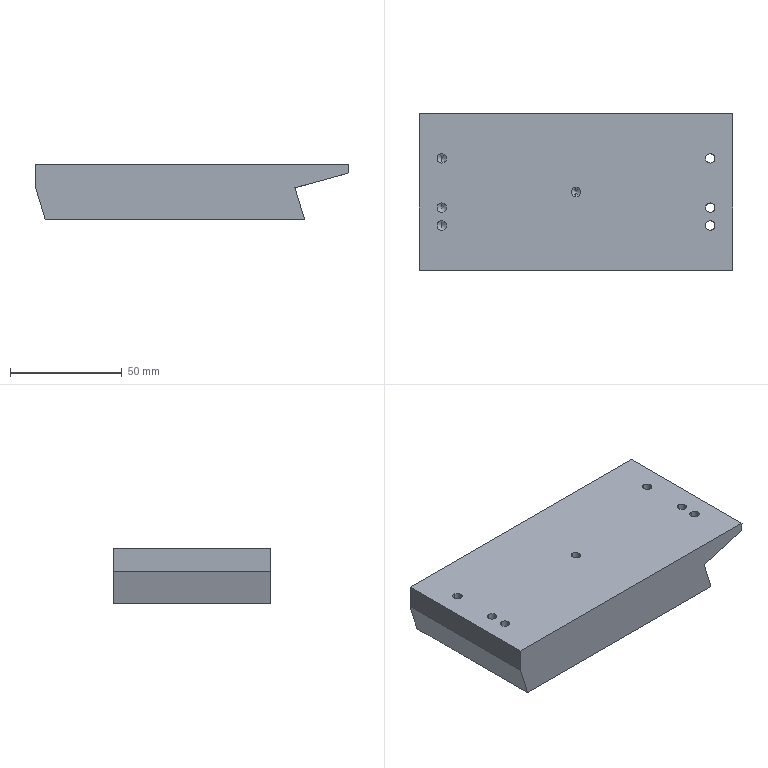Component | SolidWorks | FlatFeed-1_Part77-1 | 1 solid | 31 faces | box 140 x 70 x 25 mm | volume 214310 mm3 | cylinder 14 | plane 9 | cone 8 | commonest cylinder face diameters 4.2 x14
build123d program:
from build123d import *

# Parameters (mm, degrees)
EXTRUDE1_START        = -67.09
EXTRUDE1_DEPTH        = 70
M5_TAPPED_HOLE1_D     = 4.2
M5_TAPPED_HOLE1_DEPTH = 12.4
M5_TAPPED_HOLE1_TIP   = 1.262


with BuildPart() as part:
    # Sketch5 → Extrude1 (new body)
    with BuildSketch(Plane.XY.offset(EXTRUDE1_START)):
        Polygon((-988.993, 8051.776), (-988.993, 8047.776), (-964.993, 8041.132), (-969.382, 8026.776), (-853.382, 8026.776), (-848.993, 8041.132), (-848.993, 8051.776), align=None)
    extrude(amount=-EXTRUDE1_DEPTH)

    # M5 Tapped Hole1
    with Locations(Plane(origin=(0, 8051.776, 0), x_dir=(-1, 0, 0), z_dir=(0, 1, 0))):
        with Locations((978.993, -117.09), (978.993, -87.09), (858.993, -87.09), (858.993, -117.09), (978.993, -109.09), (918.993, -102.09), (858.993, -109.09)):
            Hole(M5_TAPPED_HOLE1_D / 2, depth=M5_TAPPED_HOLE1_DEPTH)
            with Locations((0, 0, -(M5_TAPPED_HOLE1_DEPTH + M5_TAPPED_HOLE1_TIP / 2))):  # 118° drill point
                Cone(0, M5_TAPPED_HOLE1_D / 2, M5_TAPPED_HOLE1_TIP, mode=Mode.SUBTRACT)


solid = part.part

# Placed as in the assembly
solid = solid.moved(Location((-740.399, -116.087, -7280.776), (-90, 0, 180)))
STEP:
#1=CARTESIAN_POINT('',(9.393,-9.097,30.088));
#2=VERTEX_POINT('',#1);
#3=CARTESIAN_POINT('',(9.393,-9.263,30.088));
#4=VERTEX_POINT('',#3);
#5=CARTESIAN_POINT('',(9.393,-9.097,30.088));
#6=CARTESIAN_POINT('',(9.559,-9.097,30.134));
#7=CARTESIAN_POINT('',(9.559,-9.263,30.134));
#8=CARTESIAN_POINT('',(9.393,-9.263,30.088));
#9=(BOUNDED_CURVE()B_SPLINE_CURVE(3,(#5,#6,#7,#8),.UNSPECIFIED.,.F.,.T.)B_SPLINE_CURVE_WITH_KNOTS((4,4),(4.712,7.854),.UNSPECIFIED.)CURVE()GEOMETRIC_REPRESENTATION_ITEM()RATIONAL_B_SPLINE_CURVE((1.,0.3333,0.3333,1.))REPRESENTATION_ITEM(''));
#10=EDGE_CURVE('',#2,#4,#9,.T.);
#11=ORIENTED_EDGE('',*,*,#10,.T.);
#12=CARTESIAN_POINT('',(9.393,-9.263,30.354));
#13=VERTEX_POINT('',#12);
#14=CARTESIAN_POINT('',(9.393,-9.263,30.354));
#15=DIRECTION('',(-0.,0.,1.));
#16=VECTOR('',#15,39.37);
#17=LINE('',#14,#16);
#18=EDGE_CURVE('',#4,#13,#17,.T.);
#19=ORIENTED_EDGE('',*,*,#18,.T.);
#20=CARTESIAN_POINT('',(9.393,-9.097,30.354));
#21=VERTEX_POINT('',#20);
#22=CARTESIAN_POINT('',(9.393,-9.18,30.354));
#23=DIRECTION('',(-0.,0.,1.));
#24=DIRECTION('',(0.,1.,0.));
#25=AXIS2_PLACEMENT_3D('',#22,#23,#24);
#26=CIRCLE('',#25,0.08268);
#27=EDGE_CURVE('',#13,#21,#26,.T.);
#28=ORIENTED_EDGE('',*,*,#27,.T.);
#29=CARTESIAN_POINT('',(9.393,-9.097,30.354));
#30=DIRECTION('',(-0.,0.,1.));
#31=VECTOR('',#30,39.37);
#32=LINE('',#29,#31);
#33=EDGE_CURVE('',#2,#21,#32,.T.);
#34=ORIENTED_EDGE('',*,*,#33,.F.);
#35=EDGE_LOOP('',(#11,#19,#28,#34));
#36=FACE_OUTER_BOUND('',#35,.T.);
#37=CARTESIAN_POINT('',(9.393,-9.18,30.354));
#38=DIRECTION('',(-0.,0.,1.));
#39=DIRECTION('',(0.,1.,0.));
#40=AXIS2_PLACEMENT_3D('',#37,#38,#39);
#41=CYLINDRICAL_SURFACE('',#40,0.08268);
#42=ADVANCED_FACE('',(#36),#41,.F.);
#43=CARTESIAN_POINT('',(9.393,-7.916,30.088));
#44=VERTEX_POINT('',#43);
#45=CARTESIAN_POINT('',(9.393,-8.082,30.088));
#46=VERTEX_POINT('',#45);
#47=CARTESIAN_POINT('',(9.393,-7.916,30.088));
#48=CARTESIAN_POINT('',(9.559,-7.916,30.134));
#49=CARTESIAN_POINT('',(9.559,-8.082,30.134));
#50=CARTESIAN_POINT('',(9.393,-8.082,30.088));
#51=(BOUNDED_CURVE()B_SPLINE_CURVE(3,(#47,#48,#49,#50),.UNSPECIFIED.,.F.,.T.)B_SPLINE_CURVE_WITH_KNOTS((4,4),(4.712,7.854),.UNSPECIFIED.)CURVE()GEOMETRIC_REPRESENTATION_ITEM()RATIONAL_B_SPLINE_CURVE((1.,0.3333,0.3333,1.))REPRESENTATION_ITEM(''));
#52=EDGE_CURVE('',#44,#46,#51,.T.);
#53=ORIENTED_EDGE('',*,*,#52,.T.);
#54=CARTESIAN_POINT('',(9.393,-8.082,30.354));
#55=VERTEX_POINT('',#54);
#56=CARTESIAN_POINT('',(9.393,-8.082,30.354));
#57=DIRECTION('',(-0.,0.,1.));
#58=VECTOR('',#57,39.37);
#59=LINE('',#56,#58);
#60=EDGE_CURVE('',#46,#55,#59,.T.);
#61=ORIENTED_EDGE('',*,*,#60,.T.);
#62=CARTESIAN_POINT('',(9.393,-7.916,30.354));
#63=VERTEX_POINT('',#62);
#64=CARTESIAN_POINT('',(9.393,-7.999,30.354));
#65=DIRECTION('',(-0.,0.,1.));
#66=DIRECTION('',(0.,1.,0.));
#67=AXIS2_PLACEMENT_3D('',#64,#65,#66);
#68=CIRCLE('',#67,0.08268);
#69=EDGE_CURVE('',#55,#63,#68,.T.);
#70=ORIENTED_EDGE('',*,*,#69,.T.);
#71=CARTESIAN_POINT('',(9.393,-7.916,30.354));
#72=DIRECTION('',(-0.,0.,1.));
#73=VECTOR('',#72,39.37);
#74=LINE('',#71,#73);
#75=EDGE_CURVE('',#44,#63,#74,.T.);
#76=ORIENTED_EDGE('',*,*,#75,.F.);
#77=EDGE_LOOP('',(#53,#61,#70,#76));
#78=FACE_OUTER_BOUND('',#77,.T.);
#79=CARTESIAN_POINT('',(9.393,-7.999,30.354));
#80=DIRECTION('',(-0.,0.,1.));
#81=DIRECTION('',(0.,1.,0.));
#82=AXIS2_PLACEMENT_3D('',#79,#80,#81);
#83=CYLINDRICAL_SURFACE('',#82,0.08268);
#84=ADVANCED_FACE('',(#78),#83,.F.);
#85=CARTESIAN_POINT('',(4.669,-8.082,29.866));
#86=VERTEX_POINT('',#85);
#87=CARTESIAN_POINT('',(4.669,-7.916,29.866));
#88=VERTEX_POINT('',#87);
#89=CARTESIAN_POINT('',(4.669,-7.999,29.866));
#90=DIRECTION('',(-0.,0.,1.));
#91=DIRECTION('',(0.,1.,0.));
#92=AXIS2_PLACEMENT_3D('',#89,#90,#91);
#93=CIRCLE('',#92,0.08268);
#94=EDGE_CURVE('',#86,#88,#93,.T.);
#95=ORIENTED_EDGE('',*,*,#94,.F.);
#96=CARTESIAN_POINT('',(4.669,-8.082,30.354));
#97=VERTEX_POINT('',#96);
#98=CARTESIAN_POINT('',(4.669,-8.082,30.354));
#99=DIRECTION('',(-0.,0.,1.));
#100=VECTOR('',#99,39.37);
#101=LINE('',#98,#100);
#102=EDGE_CURVE('',#86,#97,#101,.T.);
#103=ORIENTED_EDGE('',*,*,#102,.T.);
#104=CARTESIAN_POINT('',(4.669,-7.916,30.354));
#105=VERTEX_POINT('',#104);
#106=CARTESIAN_POINT('',(4.669,-7.999,30.354));
#107=DIRECTION('',(-0.,0.,1.));
#108=DIRECTION('',(0.,1.,0.));
#109=AXIS2_PLACEMENT_3D('',#106,#107,#108);
#110=CIRCLE('',#109,0.08268);
#111=EDGE_CURVE('',#97,#105,#110,.T.);
#112=ORIENTED_EDGE('',*,*,#111,.T.);
#113=CARTESIAN_POINT('',(4.669,-7.916,30.354));
#114=DIRECTION('',(-0.,0.,1.));
#115=VECTOR('',#114,39.37);
#116=LINE('',#113,#115);
#117=EDGE_CURVE('',#88,#105,#116,.T.);
#118=ORIENTED_EDGE('',*,*,#117,.F.);
#119=EDGE_LOOP('',(#95,#103,#112,#118));
#120=FACE_OUTER_BOUND('',#119,.T.);
#121=CARTESIAN_POINT('',(4.669,-7.999,30.354));
#122=DIRECTION('',(-0.,0.,1.));
#123=DIRECTION('',(0.,1.,0.));
#124=AXIS2_PLACEMENT_3D('',#121,#122,#123);
#125=CYLINDRICAL_SURFACE('',#124,0.08268);
#126=ADVANCED_FACE('',(#120),#125,.F.);
#127=CARTESIAN_POINT('',(4.669,-7.999,29.816));
#128=VERTEX_POINT('',#127);
#129=CARTESIAN_POINT('',(4.669,-7.916,29.866));
#130=DIRECTION('',(-0.,0.8572,0.515));
#131=VECTOR('',#130,39.37);
#132=LINE('',#129,#131);
#133=EDGE_CURVE('',#128,#88,#132,.T.);
#134=ORIENTED_EDGE('',*,*,#133,.F.);
#135=CARTESIAN_POINT('',(4.669,-8.082,29.866));
#136=DIRECTION('',(-0.,-0.8572,0.515));
#137=VECTOR('',#136,39.37);
#138=LINE('',#135,#137);
#139=EDGE_CURVE('',#128,#86,#138,.T.);
#140=ORIENTED_EDGE('',*,*,#139,.T.);
#141=ORIENTED_EDGE('',*,*,#94,.T.);
#142=EDGE_LOOP('',(#134,#140,#141));
#143=FACE_OUTER_BOUND('',#142,.T.);
#144=CARTESIAN_POINT('',(4.669,-7.999,29.866));
#145=DIRECTION('',(-0.,0.,1.));
#146=DIRECTION('',(0.,1.,0.));
#147=AXIS2_PLACEMENT_3D('',#144,#145,#146);
#148=CONICAL_SURFACE('',#147,0.08268,1.03);
#149=ADVANCED_FACE('',(#143),#148,.F.);
#150=CARTESIAN_POINT('',(4.669,-9.263,29.866));
#151=VERTEX_POINT('',#150);
#152=CARTESIAN_POINT('',(4.669,-9.097,29.866));
#153=VERTEX_POINT('',#152);
#154=CARTESIAN_POINT('',(4.669,-9.18,29.866));
#155=DIRECTION('',(-0.,0.,1.));
#156=DIRECTION('',(0.,1.,0.));
#157=AXIS2_PLACEMENT_3D('',#154,#155,#156);
#158=CIRCLE('',#157,0.08268);
#159=EDGE_CURVE('',#151,#153,#158,.T.);
#160=ORIENTED_EDGE('',*,*,#159,.F.);
#161=CARTESIAN_POINT('',(4.669,-9.263,30.354));
#162=VERTEX_POINT('',#161);
#163=CARTESIAN_POINT('',(4.669,-9.263,30.354));
#164=DIRECTION('',(-0.,0.,1.));
#165=VECTOR('',#164,39.37);
#166=LINE('',#163,#165);
#167=EDGE_CURVE('',#151,#162,#166,.T.);
#168=ORIENTED_EDGE('',*,*,#167,.T.);
#169=CARTESIAN_POINT('',(4.669,-9.097,30.354));
#170=VERTEX_POINT('',#169);
#171=CARTESIAN_POINT('',(4.669,-9.18,30.354));
#172=DIRECTION('',(-0.,0.,1.));
#173=DIRECTION('',(0.,1.,0.));
#174=AXIS2_PLACEMENT_3D('',#171,#172,#173);
#175=CIRCLE('',#174,0.08268);
#176=EDGE_CURVE('',#162,#170,#175,.T.);
#177=ORIENTED_EDGE('',*,*,#176,.T.);
#178=CARTESIAN_POINT('',(4.669,-9.097,30.354));
#179=DIRECTION('',(-0.,0.,1.));
#180=VECTOR('',#179,39.37);
#181=LINE('',#178,#180);
#182=EDGE_CURVE('',#153,#170,#181,.T.);
#183=ORIENTED_EDGE('',*,*,#182,.F.);
#184=EDGE_LOOP('',(#160,#168,#177,#183));
#185=FACE_OUTER_BOUND('',#184,.T.);
#186=CARTESIAN_POINT('',(4.669,-9.18,30.354));
#187=DIRECTION('',(-0.,0.,1.));
#188=DIRECTION('',(0.,1.,0.));
#189=AXIS2_PLACEMENT_3D('',#186,#187,#188);
#190=CYLINDRICAL_SURFACE('',#189,0.08268);
#191=ADVANCED_FACE('',(#185),#190,.F.);
#192=CARTESIAN_POINT('',(4.669,-9.18,29.816));
#193=VERTEX_POINT('',#192);
#194=CARTESIAN_POINT('',(4.669,-9.097,29.866));
#195=DIRECTION('',(-0.,0.8572,0.515));
#196=VECTOR('',#195,39.37);
#197=LINE('',#194,#196);
#198=EDGE_CURVE('',#193,#153,#197,.T.);
#199=ORIENTED_EDGE('',*,*,#198,.F.);
#200=CARTESIAN_POINT('',(4.669,-9.263,29.866));
#201=DIRECTION('',(-0.,-0.8572,0.515));
#202=VECTOR('',#201,39.37);
#203=LINE('',#200,#202);
#204=EDGE_CURVE('',#193,#151,#203,.T.);
#205=ORIENTED_EDGE('',*,*,#204,.T.);
#206=ORIENTED_EDGE('',*,*,#159,.T.);
#207=EDGE_LOOP('',(#199,#205,#206));
#208=FACE_OUTER_BOUND('',#207,.T.);
#209=CARTESIAN_POINT('',(4.669,-9.18,29.866));
#210=DIRECTION('',(-0.,0.,1.));
#211=DIRECTION('',(0.,1.,0.));
#212=AXIS2_PLACEMENT_3D('',#209,#210,#211);
#213=CONICAL_SURFACE('',#212,0.08268,1.03);
#214=ADVANCED_FACE('',(#208),#213,.F.);
#215=CARTESIAN_POINT('',(9.393,-8.783,30.088));
#216=VERTEX_POINT('',#215);
#217=CARTESIAN_POINT('',(9.393,-8.948,30.088));
#218=VERTEX_POINT('',#217);
#219=CARTESIAN_POINT('',(9.393,-8.783,30.088));
#220=CARTESIAN_POINT('',(9.559,-8.783,30.134));
#221=CARTESIAN_POINT('',(9.559,-8.948,30.134));
#222=CARTESIAN_POINT('',(9.393,-8.948,30.088));
#223=(BOUNDED_CURVE()B_SPLINE_CURVE(3,(#219,#220,#221,#222),.UNSPECIFIED.,.F.,.T.)B_SPLINE_CURVE_WITH_KNOTS((4,4),(4.712,7.854),.UNSPECIFIED.)CURVE()GEOMETRIC_REPRESENTATION_ITEM()RATIONAL_B_SPLINE_CURVE((1.,0.3333,0.3333,1.))REPRESENTATION_ITEM(''));
#224=EDGE_CURVE('',#216,#218,#223,.T.);
#225=ORIENTED_EDGE('',*,*,#224,.T.);
#226=CARTESIAN_POINT('',(9.393,-8.948,30.354));
#227=VERTEX_POINT('',#226);
#228=CARTESIAN_POINT('',(9.393,-8.948,30.354));
#229=DIRECTION('',(-0.,0.,1.));
#230=VECTOR('',#229,39.37);
#231=LINE('',#228,#230);
#232=EDGE_CURVE('',#218,#227,#231,.T.);
#233=ORIENTED_EDGE('',*,*,#232,.T.);
#234=CARTESIAN_POINT('',(9.393,-8.783,30.354));
#235=VERTEX_POINT('',#234);
#236=CARTESIAN_POINT('',(9.393,-8.865,30.354));
#237=DIRECTION('',(-0.,0.,1.));
#238=DIRECTION('',(0.,1.,0.));
#239=AXIS2_PLACEMENT_3D('',#236,#237,#238);
#240=CIRCLE('',#239,0.08268);
#241=EDGE_CURVE('',#227,#235,#240,.T.);
#242=ORIENTED_EDGE('',*,*,#241,.T.);
#243=CARTESIAN_POINT('',(9.393,-8.783,30.354));
#244=DIRECTION('',(-0.,0.,1.));
#245=VECTOR('',#244,39.37);
#246=LINE('',#243,#245);
#247=EDGE_CURVE('',#216,#235,#246,.T.);
#248=ORIENTED_EDGE('',*,*,#247,.F.);
#249=EDGE_LOOP('',(#225,#233,#242,#248));
#250=FACE_OUTER_BOUND('',#249,.T.);
#251=CARTESIAN_POINT('',(9.393,-8.865,30.354));
#252=DIRECTION('',(-0.,0.,1.));
#253=DIRECTION('',(0.,1.,0.));
#254=AXIS2_PLACEMENT_3D('',#251,#252,#253);
#255=CYLINDRICAL_SURFACE('',#254,0.08268);
#256=ADVANCED_FACE('',(#250),#255,.F.);
#257=CARTESIAN_POINT('',(7.031,-8.672,29.866));
#258=VERTEX_POINT('',#257);
#259=CARTESIAN_POINT('',(7.031,-8.507,29.866));
#260=VERTEX_POINT('',#259);
#261=CARTESIAN_POINT('',(7.031,-8.59,29.866));
#262=DIRECTION('',(-0.,0.,1.));
#263=DIRECTION('',(0.,1.,0.));
#264=AXIS2_PLACEMENT_3D('',#261,#262,#263);
#265=CIRCLE('',#264,0.08268);
#266=EDGE_CURVE('',#258,#260,#265,.T.);
#267=ORIENTED_EDGE('',*,*,#266,.F.);
#268=CARTESIAN_POINT('',(7.031,-8.672,30.354));
#269=VERTEX_POINT('',#268);
#270=CARTESIAN_POINT('',(7.031,-8.672,30.354));
#271=DIRECTION('',(-0.,0.,1.));
#272=VECTOR('',#271,39.37);
#273=LINE('',#270,#272);
#274=EDGE_CURVE('',#258,#269,#273,.T.);
#275=ORIENTED_EDGE('',*,*,#274,.T.);
#276=CARTESIAN_POINT('',(7.031,-8.507,30.354));
#277=VERTEX_POINT('',#276);
#278=CARTESIAN_POINT('',(7.031,-8.59,30.354));
#279=DIRECTION('',(-0.,0.,1.));
#280=DIRECTION('',(0.,1.,0.));
#281=AXIS2_PLACEMENT_3D('',#278,#279,#280);
#282=CIRCLE('',#281,0.08268);
#283=EDGE_CURVE('',#269,#277,#282,.T.);
#284=ORIENTED_EDGE('',*,*,#283,.T.);
#285=CARTESIAN_POINT('',(7.031,-8.507,30.354));
#286=DIRECTION('',(-0.,0.,1.));
#287=VECTOR('',#286,39.37);
#288=LINE('',#285,#287);
#289=EDGE_CURVE('',#260,#277,#288,.T.);
#290=ORIENTED_EDGE('',*,*,#289,.F.);
#291=EDGE_LOOP('',(#267,#275,#284,#290));
#292=FACE_OUTER_BOUND('',#291,.T.);
#293=CARTESIAN_POINT('',(7.031,-8.59,30.354));
#294=DIRECTION('',(-0.,0.,1.));
#295=DIRECTION('',(0.,1.,0.));
#296=AXIS2_PLACEMENT_3D('',#293,#294,#295);
#297=CYLINDRICAL_SURFACE('',#296,0.08268);
#298=ADVANCED_FACE('',(#292),#297,.F.);
#299=CARTESIAN_POINT('',(7.031,-8.59,29.816));
#300=VERTEX_POINT('',#299);
#301=CARTESIAN_POINT('',(7.031,-8.507,29.866));
#302=DIRECTION('',(-0.,0.8572,0.515));
#303=VECTOR('',#302,39.37);
#304=LINE('',#301,#303);
#305=EDGE_CURVE('',#300,#260,#304,.T.);
#306=ORIENTED_EDGE('',*,*,#305,.F.);
#307=CARTESIAN_POINT('',(7.031,-8.672,29.866));
#308=DIRECTION('',(-0.,-0.8572,0.515));
#309=VECTOR('',#308,39.37);
#310=LINE('',#307,#309);
#311=EDGE_CURVE('',#300,#258,#310,.T.);
#312=ORIENTED_EDGE('',*,*,#311,.T.);
#313=ORIENTED_EDGE('',*,*,#266,.T.);
#314=EDGE_LOOP('',(#306,#312,#313));
#315=FACE_OUTER_BOUND('',#314,.T.);
#316=CARTESIAN_POINT('',(7.031,-8.59,29.866));
#317=DIRECTION('',(-0.,0.,1.));
#318=DIRECTION('',(0.,1.,0.));
#319=AXIS2_PLACEMENT_3D('',#316,#317,#318);
#320=CONICAL_SURFACE('',#319,0.08268,1.03);
#321=ADVANCED_FACE('',(#315),#320,.F.);
#322=CARTESIAN_POINT('',(4.669,-8.948,29.866));
#323=VERTEX_POINT('',#322);
#324=CARTESIAN_POINT('',(4.669,-8.783,29.866));
#325=VERTEX_POINT('',#324);
#326=CARTESIAN_POINT('',(4.669,-8.865,29.866));
#327=DIRECTION('',(-0.,0.,1.));
#328=DIRECTION('',(0.,1.,0.));
#329=AXIS2_PLACEMENT_3D('',#326,#327,#328);
#330=CIRCLE('',#329,0.08268);
#331=EDGE_CURVE('',#323,#325,#330,.T.);
#332=ORIENTED_EDGE('',*,*,#331,.F.);
#333=CARTESIAN_POINT('',(4.669,-8.948,30.354));
#334=VERTEX_POINT('',#333);
#335=CARTESIAN_POINT('',(4.669,-8.948,30.354));
#336=DIRECTION('',(-0.,0.,1.));
#337=VECTOR('',#336,39.37);
#338=LINE('',#335,#337);
#339=EDGE_CURVE('',#323,#334,#338,.T.);
#340=ORIENTED_EDGE('',*,*,#339,.T.);
#341=CARTESIAN_POINT('',(4.669,-8.783,30.354));
#342=VERTEX_POINT('',#341);
#343=CARTESIAN_POINT('',(4.669,-8.865,30.354));
#344=DIRECTION('',(-0.,0.,1.));
#345=DIRECTION('',(0.,1.,0.));
#346=AXIS2_PLACEMENT_3D('',#343,#344,#345);
#347=CIRCLE('',#346,0.08268);
#348=EDGE_CURVE('',#334,#342,#347,.T.);
#349=ORIENTED_EDGE('',*,*,#348,.T.);
#350=CARTESIAN_POINT('',(4.669,-8.783,30.354));
#351=DIRECTION('',(-0.,0.,1.));
#352=VECTOR('',#351,39.37);
#353=LINE('',#350,#352);
#354=EDGE_CURVE('',#325,#342,#353,.T.);
#355=ORIENTED_EDGE('',*,*,#354,.F.);
#356=EDGE_LOOP('',(#332,#340,#349,#355));
#357=FACE_OUTER_BOUND('',#356,.T.);
#358=CARTESIAN_POINT('',(4.669,-8.865,30.354));
#359=DIRECTION('',(-0.,0.,1.));
#360=DIRECTION('',(0.,1.,0.));
#361=AXIS2_PLACEMENT_3D('',#358,#359,#360);
#362=CYLINDRICAL_SURFACE('',#361,0.08268);
#363=ADVANCED_FACE('',(#357),#362,.F.);
#364=CARTESIAN_POINT('',(4.669,-8.865,29.816));
#365=VERTEX_POINT('',#364);
#366=CARTESIAN_POINT('',(4.669,-8.783,29.866));
#367=DIRECTION('',(-0.,0.8572,0.515));
#368=VECTOR('',#367,39.37);
#369=LINE('',#366,#368);
#370=EDGE_CURVE('',#365,#325,#369,.T.);
#371=ORIENTED_EDGE('',*,*,#370,.F.);
#372=CARTESIAN_POINT('',(4.669,-8.948,29.866));
#373=DIRECTION('',(-0.,-0.8572,0.515));
#374=VECTOR('',#373,39.37);
#375=LINE('',#372,#374);
#376=EDGE_CURVE('',#365,#323,#375,.T.);
#377=ORIENTED_EDGE('',*,*,#376,.T.);
#378=ORIENTED_EDGE('',*,*,#331,.T.);
#379=EDGE_LOOP('',(#371,#377,#378));
#380=FACE_OUTER_BOUND('',#379,.T.);
#381=CARTESIAN_POINT('',(4.669,-8.865,29.866));
#382=DIRECTION('',(-0.,0.,1.));
#383=DIRECTION('',(0.,1.,0.));
#384=AXIS2_PLACEMENT_3D('',#381,#382,#383);
#385=CONICAL_SURFACE('',#384,0.08268,1.03);
#386=ADVANCED_FACE('',(#380),#385,.F.);
#387=CARTESIAN_POINT('',(4.448,-7.212,29.37));
#388=VERTEX_POINT('',#387);
#389=CARTESIAN_POINT('',(4.275,-7.212,29.935));
#390=VERTEX_POINT('',#389);
#391=CARTESIAN_POINT('',(4.275,-7.212,29.935));
#392=DIRECTION('',(-0.2924,0.,0.9563));
#393=VECTOR('',#392,39.37);
#394=LINE('',#391,#393);
#395=EDGE_CURVE('',#388,#390,#394,.T.);
#396=ORIENTED_EDGE('',*,*,#395,.F.);
#397=CARTESIAN_POINT('',(4.448,-9.968,29.37));
#398=VERTEX_POINT('',#397);
#399=CARTESIAN_POINT('',(4.448,-9.968,29.37));
#400=DIRECTION('',(-0.,1.,-0.));
#401=VECTOR('',#400,39.37);
#402=LINE('',#399,#401);
#403=EDGE_CURVE('',#398,#388,#402,.T.);
#404=ORIENTED_EDGE('',*,*,#403,.F.);
#405=CARTESIAN_POINT('',(4.275,-9.968,29.935));
#406=VERTEX_POINT('',#405);
#407=CARTESIAN_POINT('',(4.275,-9.968,29.935));
#408=DIRECTION('',(-0.2924,0.,0.9563));
#409=VECTOR('',#408,39.37);
#410=LINE('',#407,#409);
#411=EDGE_CURVE('',#398,#406,#410,.T.);
#412=ORIENTED_EDGE('',*,*,#411,.T.);
#413=CARTESIAN_POINT('',(4.275,-9.968,29.935));
#414=DIRECTION('',(-0.,1.,-0.));
#415=VECTOR('',#414,39.37);
#416=LINE('',#413,#415);
#417=EDGE_CURVE('',#406,#390,#416,.T.);
#418=ORIENTED_EDGE('',*,*,#417,.T.);
#419=EDGE_LOOP('',(#396,#404,#412,#418));
#420=FACE_OUTER_BOUND('',#419,.T.);
#421=CARTESIAN_POINT('',(4.275,-9.968,29.935));
#422=DIRECTION('',(-0.9563,-0.,-0.2924));
#423=DIRECTION('',(-0.2924,0.,0.9563));
#424=AXIS2_PLACEMENT_3D('',#421,#422,#423);
#425=PLANE('',#424);
#426=ADVANCED_FACE('',(#420),#425,.T.);
#427=CARTESIAN_POINT('',(9.015,-7.212,29.37));
#428=VERTEX_POINT('',#427);
#429=CARTESIAN_POINT('',(4.448,-7.212,29.37));
#430=DIRECTION('',(-1.,-0.,-0.));
#431=VECTOR('',#430,39.37);
#432=LINE('',#429,#431);
#433=EDGE_CURVE('',#428,#388,#432,.T.);
#434=ORIENTED_EDGE('',*,*,#433,.F.);
#435=CARTESIAN_POINT('',(9.015,-9.968,29.37));
#436=VERTEX_POINT('',#435);
#437=CARTESIAN_POINT('',(9.015,-9.968,29.37));
#438=DIRECTION('',(-0.,1.,-0.));
#439=VECTOR('',#438,39.37);
#440=LINE('',#437,#439);
#441=EDGE_CURVE('',#436,#428,#440,.T.);
#442=ORIENTED_EDGE('',*,*,#441,.F.);
#443=CARTESIAN_POINT('',(4.448,-9.968,29.37));
#444=DIRECTION('',(-1.,-0.,-0.));
#445=VECTOR('',#444,39.37);
#446=LINE('',#443,#445);
#447=EDGE_CURVE('',#436,#398,#446,.T.);
#448=ORIENTED_EDGE('',*,*,#447,.T.);
#449=ORIENTED_EDGE('',*,*,#403,.T.);
#450=EDGE_LOOP('',(#434,#442,#448,#449));
#451=FACE_OUTER_BOUND('',#450,.T.);
#452=CARTESIAN_POINT('',(4.448,-9.968,29.37));
#453=DIRECTION('',(0.,-0.,-1.));
#454=DIRECTION('',(-1.,-0.,-0.));
#455=AXIS2_PLACEMENT_3D('',#452,#453,#454);
#456=PLANE('',#455);
#457=ADVANCED_FACE('',(#451),#456,.T.);
#458=CARTESIAN_POINT('',(8.842,-7.212,29.935));
#459=VERTEX_POINT('',#458);
#460=CARTESIAN_POINT('',(9.015,-7.212,29.37));
#461=DIRECTION('',(0.2924,-0.,-0.9563));
#462=VECTOR('',#461,39.37);
#463=LINE('',#460,#462);
#464=EDGE_CURVE('',#459,#428,#463,.T.);
#465=ORIENTED_EDGE('',*,*,#464,.F.);
#466=CARTESIAN_POINT('',(8.842,-9.968,29.935));
#467=VERTEX_POINT('',#466);
#468=CARTESIAN_POINT('',(8.842,-9.968,29.935));
#469=DIRECTION('',(-0.,1.,-0.));
#470=VECTOR('',#469,39.37);
#471=LINE('',#468,#470);
#472=EDGE_CURVE('',#467,#459,#471,.T.);
#473=ORIENTED_EDGE('',*,*,#472,.F.);
#474=CARTESIAN_POINT('',(9.015,-9.968,29.37));
#475=DIRECTION('',(0.2924,-0.,-0.9563));
#476=VECTOR('',#475,39.37);
#477=LINE('',#474,#476);
#478=EDGE_CURVE('',#467,#436,#477,.T.);
#479=ORIENTED_EDGE('',*,*,#478,.T.);
#480=ORIENTED_EDGE('',*,*,#441,.T.);
#481=EDGE_LOOP('',(#465,#473,#479,#480));
#482=FACE_OUTER_BOUND('',#481,.T.);
#483=CARTESIAN_POINT('',(9.015,-9.968,29.37));
#484=DIRECTION('',(0.9563,0.,0.2924));
#485=DIRECTION('',(0.2924,-0.,-0.9563));
#486=AXIS2_PLACEMENT_3D('',#483,#484,#485);
#487=PLANE('',#486);
#488=ADVANCED_FACE('',(#482),#487,.T.);
#489=ORIENTED_EDGE('',*,*,#10,.F.);
#490=CARTESIAN_POINT('',(9.393,-9.263,30.088));
#491=CARTESIAN_POINT('',(9.228,-9.263,30.042));
#492=CARTESIAN_POINT('',(9.228,-9.097,30.042));
#493=CARTESIAN_POINT('',(9.393,-9.097,30.088));
#494=(BOUNDED_CURVE()B_SPLINE_CURVE(3,(#490,#491,#492,#493),.UNSPECIFIED.,.F.,.T.)B_SPLINE_CURVE_WITH_KNOTS((4,4),(1.571,4.712),.UNSPECIFIED.)CURVE()GEOMETRIC_REPRESENTATION_ITEM()RATIONAL_B_SPLINE_CURVE((1.,0.3333,0.3333,1.))REPRESENTATION_ITEM(''));
#495=EDGE_CURVE('',#4,#2,#494,.T.);
#496=ORIENTED_EDGE('',*,*,#495,.F.);
#497=EDGE_LOOP('',(#489,#496));
#498=FACE_BOUND('',#497,.T.);
#499=ORIENTED_EDGE('',*,*,#52,.F.);
#500=CARTESIAN_POINT('',(9.393,-8.082,30.088));
#501=CARTESIAN_POINT('',(9.228,-8.082,30.042));
#502=CARTESIAN_POINT('',(9.228,-7.916,30.042));
#503=CARTESIAN_POINT('',(9.393,-7.916,30.088));
#504=(BOUNDED_CURVE()B_SPLINE_CURVE(3,(#500,#501,#502,#503),.UNSPECIFIED.,.F.,.T.)B_SPLINE_CURVE_WITH_KNOTS((4,4),(1.571,4.712),.UNSPECIFIED.)CURVE()GEOMETRIC_REPRESENTATION_ITEM()RATIONAL_B_SPLINE_CURVE((1.,0.3333,0.3333,1.))REPRESENTATION_ITEM(''));
#505=EDGE_CURVE('',#46,#44,#504,.T.);
#506=ORIENTED_EDGE('',*,*,#505,.F.);
#507=EDGE_LOOP('',(#499,#506));
#508=FACE_BOUND('',#507,.T.);
#509=ORIENTED_EDGE('',*,*,#224,.F.);
#510=CARTESIAN_POINT('',(9.393,-8.948,30.088));
#511=CARTESIAN_POINT('',(9.228,-8.948,30.042));
#512=CARTESIAN_POINT('',(9.228,-8.783,30.042));
#513=CARTESIAN_POINT('',(9.393,-8.783,30.088));
#514=(BOUNDED_CURVE()B_SPLINE_CURVE(3,(#510,#511,#512,#513),.UNSPECIFIED.,.F.,.T.)B_SPLINE_CURVE_WITH_KNOTS((4,4),(1.571,4.712),.UNSPECIFIED.)CURVE()GEOMETRIC_REPRESENTATION_ITEM()RATIONAL_B_SPLINE_CURVE((1.,0.3333,0.3333,1.))REPRESENTATION_ITEM(''));
#515=EDGE_CURVE('',#218,#216,#514,.T.);
#516=ORIENTED_EDGE('',*,*,#515,.F.);
#517=EDGE_LOOP('',(#509,#516));
#518=FACE_BOUND('',#517,.T.);
#519=CARTESIAN_POINT('',(9.787,-7.212,30.197));
#520=VERTEX_POINT('',#519);
#521=CARTESIAN_POINT('',(9.787,-7.212,30.197));
#522=DIRECTION('',(-0.9637,-0.,-0.2668));
#523=VECTOR('',#522,39.37);
#524=LINE('',#521,#523);
#525=EDGE_CURVE('',#520,#459,#524,.T.);
#526=ORIENTED_EDGE('',*,*,#525,.F.);
#527=CARTESIAN_POINT('',(9.787,-9.968,30.197));
#528=VERTEX_POINT('',#527);
#529=CARTESIAN_POINT('',(9.787,-9.968,30.197));
#530=DIRECTION('',(-0.,1.,-0.));
#531=VECTOR('',#530,39.37);
#532=LINE('',#529,#531);
#533=EDGE_CURVE('',#528,#520,#532,.T.);
#534=ORIENTED_EDGE('',*,*,#533,.F.);
#535=CARTESIAN_POINT('',(9.787,-9.968,30.197));
#536=DIRECTION('',(-0.9637,-0.,-0.2668));
#537=VECTOR('',#536,39.37);
#538=LINE('',#535,#537);
#539=EDGE_CURVE('',#528,#467,#538,.T.);
#540=ORIENTED_EDGE('',*,*,#539,.T.);
#541=ORIENTED_EDGE('',*,*,#472,.T.);
#542=EDGE_LOOP('',(#526,#534,#540,#541));
#543=FACE_OUTER_BOUND('',#542,.T.);
#544=CARTESIAN_POINT('',(9.787,-9.968,30.197));
#545=DIRECTION('',(0.2668,-0.,-0.9637));
#546=DIRECTION('',(-0.9637,-0.,-0.2668));
#547=AXIS2_PLACEMENT_3D('',#544,#545,#546);
#548=PLANE('',#547);
#549=ADVANCED_FACE('',(#498,#508,#518,#543),#548,.T.);
#550=CARTESIAN_POINT('',(9.787,-7.212,30.354));
#551=VERTEX_POINT('',#550);
#552=CARTESIAN_POINT('',(9.787,-7.212,30.354));
#553=DIRECTION('',(-0.,-0.,-1.));
#554=VECTOR('',#553,39.37);
#555=LINE('',#552,#554);
#556=EDGE_CURVE('',#551,#520,#555,.T.);
#557=ORIENTED_EDGE('',*,*,#556,.F.);
#558=CARTESIAN_POINT('',(9.787,-9.968,30.354));
#559=VERTEX_POINT('',#558);
#560=CARTESIAN_POINT('',(9.787,-9.968,30.354));
#561=DIRECTION('',(-0.,1.,-0.));
#562=VECTOR('',#561,39.37);
#563=LINE('',#560,#562);
#564=EDGE_CURVE('',#559,#551,#563,.T.);
#565=ORIENTED_EDGE('',*,*,#564,.F.);
#566=CARTESIAN_POINT('',(9.787,-9.968,30.354));
#567=DIRECTION('',(-0.,-0.,-1.));
#568=VECTOR('',#567,39.37);
#569=LINE('',#566,#568);
#570=EDGE_CURVE('',#559,#528,#569,.T.);
#571=ORIENTED_EDGE('',*,*,#570,.T.);
#572=ORIENTED_EDGE('',*,*,#533,.T.);
#573=EDGE_LOOP('',(#557,#565,#571,#572));
#574=FACE_OUTER_BOUND('',#573,.T.);
#575=CARTESIAN_POINT('',(9.787,-9.968,30.354));
#576=DIRECTION('',(1.,0.,-0.));
#577=DIRECTION('',(-0.,-0.,-1.));
#578=AXIS2_PLACEMENT_3D('',#575,#576,#577);
#579=PLANE('',#578);
#580=ADVANCED_FACE('',(#574),#579,.T.);
#581=CARTESIAN_POINT('',(9.393,-9.18,30.354));
#582=DIRECTION('',(-0.,0.,1.));
#583=DIRECTION('',(0.,1.,0.));
#584=AXIS2_PLACEMENT_3D('',#581,#582,#583);
#585=CIRCLE('',#584,0.08268);
#586=EDGE_CURVE('',#21,#13,#585,.T.);
#587=ORIENTED_EDGE('',*,*,#586,.F.);
#588=ORIENTED_EDGE('',*,*,#27,.F.);
#589=EDGE_LOOP('',(#587,#588));
#590=FACE_BOUND('',#589,.T.);
#591=CARTESIAN_POINT('',(9.393,-7.999,30.354));
#592=DIRECTION('',(-0.,0.,1.));
#593=DIRECTION('',(0.,1.,0.));
#594=AXIS2_PLACEMENT_3D('',#591,#592,#593);
#595=CIRCLE('',#594,0.08268);
#596=EDGE_CURVE('',#63,#55,#595,.T.);
#597=ORIENTED_EDGE('',*,*,#596,.F.);
#598=ORIENTED_EDGE('',*,*,#69,.F.);
#599=EDGE_LOOP('',(#597,#598));
#600=FACE_BOUND('',#599,.T.);
#601=CARTESIAN_POINT('',(4.669,-7.999,30.354));
#602=DIRECTION('',(-0.,0.,1.));
#603=DIRECTION('',(0.,1.,0.));
#604=AXIS2_PLACEMENT_3D('',#601,#602,#603);
#605=CIRCLE('',#604,0.08268);
#606=EDGE_CURVE('',#105,#97,#605,.T.);
#607=ORIENTED_EDGE('',*,*,#606,.F.);
#608=ORIENTED_EDGE('',*,*,#111,.F.);
#609=EDGE_LOOP('',(#607,#608));
#610=FACE_BOUND('',#609,.T.);
#611=CARTESIAN_POINT('',(4.669,-9.18,30.354));
#612=DIRECTION('',(-0.,0.,1.));
#613=DIRECTION('',(0.,1.,0.));
#614=AXIS2_PLACEMENT_3D('',#611,#612,#613);
#615=CIRCLE('',#614,0.08268);
#616=EDGE_CURVE('',#170,#162,#615,.T.);
#617=ORIENTED_EDGE('',*,*,#616,.F.);
#618=ORIENTED_EDGE('',*,*,#176,.F.);
#619=EDGE_LOOP('',(#617,#618));
#620=FACE_BOUND('',#619,.T.);
#621=CARTESIAN_POINT('',(9.393,-8.865,30.354));
#622=DIRECTION('',(-0.,0.,1.));
#623=DIRECTION('',(0.,1.,0.));
#624=AXIS2_PLACEMENT_3D('',#621,#622,#623);
#625=CIRCLE('',#624,0.08268);
#626=EDGE_CURVE('',#235,#227,#625,.T.);
#627=ORIENTED_EDGE('',*,*,#626,.F.);
#628=ORIENTED_EDGE('',*,*,#241,.F.);
#629=EDGE_LOOP('',(#627,#628));
#630=FACE_BOUND('',#629,.T.);
#631=CARTESIAN_POINT('',(7.031,-8.59,30.354));
#632=DIRECTION('',(-0.,0.,1.));
#633=DIRECTION('',(0.,1.,0.));
#634=AXIS2_PLACEMENT_3D('',#631,#632,#633);
#635=CIRCLE('',#634,0.08268);
#636=EDGE_CURVE('',#277,#269,#635,.T.);
#637=ORIENTED_EDGE('',*,*,#636,.F.);
#638=ORIENTED_EDGE('',*,*,#283,.F.);
#639=EDGE_LOOP('',(#637,#638));
#640=FACE_BOUND('',#639,.T.);
#641=CARTESIAN_POINT('',(4.669,-8.865,30.354));
#642=DIRECTION('',(-0.,0.,1.));
#643=DIRECTION('',(0.,1.,0.));
#644=AXIS2_PLACEMENT_3D('',#641,#642,#643);
#645=CIRCLE('',#644,0.08268);
#646=EDGE_CURVE('',#342,#334,#645,.T.);
#647=ORIENTED_EDGE('',*,*,#646,.F.);
#648=ORIENTED_EDGE('',*,*,#348,.F.);
#649=EDGE_LOOP('',(#647,#648));
#650=FACE_BOUND('',#649,.T.);
#651=CARTESIAN_POINT('',(4.275,-7.212,30.354));
#652=VERTEX_POINT('',#651);
#653=CARTESIAN_POINT('',(9.787,-7.212,30.354));
#654=DIRECTION('',(1.,0.,0.));
#655=VECTOR('',#654,39.37);
#656=LINE('',#653,#655);
#657=EDGE_CURVE('',#652,#551,#656,.T.);
#658=ORIENTED_EDGE('',*,*,#657,.F.);
#659=CARTESIAN_POINT('',(4.275,-9.968,30.354));
#660=VERTEX_POINT('',#659);
#661=CARTESIAN_POINT('',(4.275,-9.968,30.354));
#662=DIRECTION('',(-0.,1.,-0.));
#663=VECTOR('',#662,39.37);
#664=LINE('',#661,#663);
#665=EDGE_CURVE('',#660,#652,#664,.T.);
#666=ORIENTED_EDGE('',*,*,#665,.F.);
#667=CARTESIAN_POINT('',(9.787,-9.968,30.354));
#668=DIRECTION('',(1.,0.,0.));
#669=VECTOR('',#668,39.37);
#670=LINE('',#667,#669);
#671=EDGE_CURVE('',#660,#559,#670,.T.);
#672=ORIENTED_EDGE('',*,*,#671,.T.);
#673=ORIENTED_EDGE('',*,*,#564,.T.);
#674=EDGE_LOOP('',(#658,#666,#672,#673));
#675=FACE_OUTER_BOUND('',#674,.T.);
#676=CARTESIAN_POINT('',(9.787,-9.968,30.354));
#677=DIRECTION('',(-0.,0.,1.));
#678=DIRECTION('',(-0.,1.,-0.));
#679=AXIS2_PLACEMENT_3D('',#676,#677,#678);
#680=PLANE('',#679);
#681=ADVANCED_FACE('',(#590,#600,#610,#620,#630,#640,#650,#675),#680,.T.);
#682=CARTESIAN_POINT('',(4.275,-7.212,30.354));
#683=DIRECTION('',(-0.,0.,1.));
#684=VECTOR('',#683,39.37);
#685=LINE('',#682,#684);
#686=EDGE_CURVE('',#390,#652,#685,.T.);
#687=ORIENTED_EDGE('',*,*,#686,.F.);
#688=ORIENTED_EDGE('',*,*,#417,.F.);
#689=CARTESIAN_POINT('',(4.275,-9.968,30.354));
#690=DIRECTION('',(-0.,0.,1.));
#691=VECTOR('',#690,39.37);
#692=LINE('',#689,#691);
#693=EDGE_CURVE('',#406,#660,#692,.T.);
#694=ORIENTED_EDGE('',*,*,#693,.T.);
#695=ORIENTED_EDGE('',*,*,#665,.T.);
#696=EDGE_LOOP('',(#687,#688,#694,#695));
#697=FACE_OUTER_BOUND('',#696,.T.);
#698=CARTESIAN_POINT('',(4.275,-9.968,30.354));
#699=DIRECTION('',(-1.,-0.,-0.));
#700=DIRECTION('',(-0.,0.,1.));
#701=AXIS2_PLACEMENT_3D('',#698,#699,#700);
#702=PLANE('',#701);
#703=ADVANCED_FACE('',(#697),#702,.T.);
#704=ORIENTED_EDGE('',*,*,#411,.F.);
#705=ORIENTED_EDGE('',*,*,#447,.F.);
#706=ORIENTED_EDGE('',*,*,#478,.F.);
#707=ORIENTED_EDGE('',*,*,#539,.F.);
#708=ORIENTED_EDGE('',*,*,#570,.F.);
#709=ORIENTED_EDGE('',*,*,#671,.F.);
#710=ORIENTED_EDGE('',*,*,#693,.F.);
#711=EDGE_LOOP('',(#704,#705,#706,#707,#708,#709,#710));
#712=FACE_OUTER_BOUND('',#711,.T.);
#713=CARTESIAN_POINT('',(4.632,-9.968,28.769));
#714=DIRECTION('',(-0.,1.,-0.));
#715=DIRECTION('',(-1.,-0.,-0.));
#716=AXIS2_PLACEMENT_3D('',#713,#714,#715);
#717=PLANE('',#716);
#718=ADVANCED_FACE('',(#712),#717,.F.);
#719=ORIENTED_EDGE('',*,*,#395,.T.);
#720=ORIENTED_EDGE('',*,*,#686,.T.);
#721=ORIENTED_EDGE('',*,*,#657,.T.);
#722=ORIENTED_EDGE('',*,*,#556,.T.);
#723=ORIENTED_EDGE('',*,*,#525,.T.);
#724=ORIENTED_EDGE('',*,*,#464,.T.);
#725=ORIENTED_EDGE('',*,*,#433,.T.);
#726=EDGE_LOOP('',(#719,#720,#721,#722,#723,#724,#725));
#727=FACE_OUTER_BOUND('',#726,.T.);
#728=CARTESIAN_POINT('',(4.632,-7.212,28.769));
#729=DIRECTION('',(-0.,1.,-0.));
#730=DIRECTION('',(-1.,-0.,-0.));
#731=AXIS2_PLACEMENT_3D('',#728,#729,#730);
#732=PLANE('',#731);
#733=ADVANCED_FACE('',(#727),#732,.T.);
#734=ORIENTED_EDGE('',*,*,#376,.F.);
#735=ORIENTED_EDGE('',*,*,#370,.T.);
#736=CARTESIAN_POINT('',(4.669,-8.865,29.866));
#737=DIRECTION('',(-0.,0.,1.));
#738=DIRECTION('',(0.,1.,0.));
#739=AXIS2_PLACEMENT_3D('',#736,#737,#738);
#740=CIRCLE('',#739,0.08268);
#741=EDGE_CURVE('',#325,#323,#740,.T.);
#742=ORIENTED_EDGE('',*,*,#741,.T.);
#743=EDGE_LOOP('',(#734,#735,#742));
#744=FACE_OUTER_BOUND('',#743,.T.);
#745=CARTESIAN_POINT('',(4.669,-8.865,29.866));
#746=DIRECTION('',(-0.,0.,1.));
#747=DIRECTION('',(0.,1.,0.));
#748=AXIS2_PLACEMENT_3D('',#745,#746,#747);
#749=CONICAL_SURFACE('',#748,0.08268,1.03);
#750=ADVANCED_FACE('',(#744),#749,.F.);
#751=ORIENTED_EDGE('',*,*,#339,.F.);
#752=ORIENTED_EDGE('',*,*,#741,.F.);
#753=ORIENTED_EDGE('',*,*,#354,.T.);
#754=ORIENTED_EDGE('',*,*,#646,.T.);
#755=EDGE_LOOP('',(#751,#752,#753,#754));
#756=FACE_OUTER_BOUND('',#755,.T.);
#757=CARTESIAN_POINT('',(4.669,-8.865,30.354));
#758=DIRECTION('',(-0.,0.,1.));
#759=DIRECTION('',(0.,1.,0.));
#760=AXIS2_PLACEMENT_3D('',#757,#758,#759);
#761=CYLINDRICAL_SURFACE('',#760,0.08268);
#762=ADVANCED_FACE('',(#756),#761,.F.);
#763=ORIENTED_EDGE('',*,*,#311,.F.);
#764=ORIENTED_EDGE('',*,*,#305,.T.);
#765=CARTESIAN_POINT('',(7.031,-8.59,29.866));
#766=DIRECTION('',(-0.,0.,1.));
#767=DIRECTION('',(0.,1.,0.));
#768=AXIS2_PLACEMENT_3D('',#765,#766,#767);
#769=CIRCLE('',#768,0.08268);
#770=EDGE_CURVE('',#260,#258,#769,.T.);
#771=ORIENTED_EDGE('',*,*,#770,.T.);
#772=EDGE_LOOP('',(#763,#764,#771));
#773=FACE_OUTER_BOUND('',#772,.T.);
#774=CARTESIAN_POINT('',(7.031,-8.59,29.866));
#775=DIRECTION('',(-0.,0.,1.));
#776=DIRECTION('',(0.,1.,0.));
#777=AXIS2_PLACEMENT_3D('',#774,#775,#776);
#778=CONICAL_SURFACE('',#777,0.08268,1.03);
#779=ADVANCED_FACE('',(#773),#778,.F.);
#780=ORIENTED_EDGE('',*,*,#274,.F.);
#781=ORIENTED_EDGE('',*,*,#770,.F.);
#782=ORIENTED_EDGE('',*,*,#289,.T.);
#783=ORIENTED_EDGE('',*,*,#636,.T.);
#784=EDGE_LOOP('',(#780,#781,#782,#783));
#785=FACE_OUTER_BOUND('',#784,.T.);
#786=CARTESIAN_POINT('',(7.031,-8.59,30.354));
#787=DIRECTION('',(-0.,0.,1.));
#788=DIRECTION('',(0.,1.,0.));
#789=AXIS2_PLACEMENT_3D('',#786,#787,#788);
#790=CYLINDRICAL_SURFACE('',#789,0.08268);
#791=ADVANCED_FACE('',(#785),#790,.F.);
#792=ORIENTED_EDGE('',*,*,#232,.F.);
#793=ORIENTED_EDGE('',*,*,#515,.T.);
#794=ORIENTED_EDGE('',*,*,#247,.T.);
#795=ORIENTED_EDGE('',*,*,#626,.T.);
#796=EDGE_LOOP('',(#792,#793,#794,#795));
#797=FACE_OUTER_BOUND('',#796,.T.);
#798=CARTESIAN_POINT('',(9.393,-8.865,30.354));
#799=DIRECTION('',(-0.,0.,1.));
#800=DIRECTION('',(0.,1.,0.));
#801=AXIS2_PLACEMENT_3D('',#798,#799,#800);
#802=CYLINDRICAL_SURFACE('',#801,0.08268);
#803=ADVANCED_FACE('',(#797),#802,.F.);
#804=ORIENTED_EDGE('',*,*,#204,.F.);
#805=ORIENTED_EDGE('',*,*,#198,.T.);
#806=CARTESIAN_POINT('',(4.669,-9.18,29.866));
#807=DIRECTION('',(-0.,0.,1.));
#808=DIRECTION('',(0.,1.,0.));
#809=AXIS2_PLACEMENT_3D('',#806,#807,#808);
#810=CIRCLE('',#809,0.08268);
#811=EDGE_CURVE('',#153,#151,#810,.T.);
#812=ORIENTED_EDGE('',*,*,#811,.T.);
#813=EDGE_LOOP('',(#804,#805,#812));
#814=FACE_OUTER_BOUND('',#813,.T.);
#815=CARTESIAN_POINT('',(4.669,-9.18,29.866));
#816=DIRECTION('',(-0.,0.,1.));
#817=DIRECTION('',(0.,1.,0.));
#818=AXIS2_PLACEMENT_3D('',#815,#816,#817);
#819=CONICAL_SURFACE('',#818,0.08268,1.03);
#820=ADVANCED_FACE('',(#814),#819,.F.);
#821=ORIENTED_EDGE('',*,*,#167,.F.);
#822=ORIENTED_EDGE('',*,*,#811,.F.);
#823=ORIENTED_EDGE('',*,*,#182,.T.);
#824=ORIENTED_EDGE('',*,*,#616,.T.);
#825=EDGE_LOOP('',(#821,#822,#823,#824));
#826=FACE_OUTER_BOUND('',#825,.T.);
#827=CARTESIAN_POINT('',(4.669,-9.18,30.354));
#828=DIRECTION('',(-0.,0.,1.));
#829=DIRECTION('',(0.,1.,0.));
#830=AXIS2_PLACEMENT_3D('',#827,#828,#829);
#831=CYLINDRICAL_SURFACE('',#830,0.08268);
#832=ADVANCED_FACE('',(#826),#831,.F.);
#833=ORIENTED_EDGE('',*,*,#139,.F.);
#834=ORIENTED_EDGE('',*,*,#133,.T.);
#835=CARTESIAN_POINT('',(4.669,-7.999,29.866));
#836=DIRECTION('',(-0.,0.,1.));
#837=DIRECTION('',(0.,1.,0.));
#838=AXIS2_PLACEMENT_3D('',#835,#836,#837);
#839=CIRCLE('',#838,0.08268);
#840=EDGE_CURVE('',#88,#86,#839,.T.);
#841=ORIENTED_EDGE('',*,*,#840,.T.);
#842=EDGE_LOOP('',(#833,#834,#841));
#843=FACE_OUTER_BOUND('',#842,.T.);
#844=CARTESIAN_POINT('',(4.669,-7.999,29.866));
#845=DIRECTION('',(-0.,0.,1.));
#846=DIRECTION('',(0.,1.,0.));
#847=AXIS2_PLACEMENT_3D('',#844,#845,#846);
#848=CONICAL_SURFACE('',#847,0.08268,1.03);
#849=ADVANCED_FACE('',(#843),#848,.F.);
#850=ORIENTED_EDGE('',*,*,#102,.F.);
#851=ORIENTED_EDGE('',*,*,#840,.F.);
#852=ORIENTED_EDGE('',*,*,#117,.T.);
#853=ORIENTED_EDGE('',*,*,#606,.T.);
#854=EDGE_LOOP('',(#850,#851,#852,#853));
#855=FACE_OUTER_BOUND('',#854,.T.);
#856=CARTESIAN_POINT('',(4.669,-7.999,30.354));
#857=DIRECTION('',(-0.,0.,1.));
#858=DIRECTION('',(0.,1.,0.));
#859=AXIS2_PLACEMENT_3D('',#856,#857,#858);
#860=CYLINDRICAL_SURFACE('',#859,0.08268);
#861=ADVANCED_FACE('',(#855),#860,.F.);
#862=ORIENTED_EDGE('',*,*,#60,.F.);
#863=ORIENTED_EDGE('',*,*,#505,.T.);
#864=ORIENTED_EDGE('',*,*,#75,.T.);
#865=ORIENTED_EDGE('',*,*,#596,.T.);
#866=EDGE_LOOP('',(#862,#863,#864,#865));
#867=FACE_OUTER_BOUND('',#866,.T.);
#868=CARTESIAN_POINT('',(9.393,-7.999,30.354));
#869=DIRECTION('',(-0.,0.,1.));
#870=DIRECTION('',(0.,1.,0.));
#871=AXIS2_PLACEMENT_3D('',#868,#869,#870);
#872=CYLINDRICAL_SURFACE('',#871,0.08268);
#873=ADVANCED_FACE('',(#867),#872,.F.);
#874=ORIENTED_EDGE('',*,*,#18,.F.);
#875=ORIENTED_EDGE('',*,*,#495,.T.);
#876=ORIENTED_EDGE('',*,*,#33,.T.);
#877=ORIENTED_EDGE('',*,*,#586,.T.);
#878=EDGE_LOOP('',(#874,#875,#876,#877));
#879=FACE_OUTER_BOUND('',#878,.T.);
#880=CARTESIAN_POINT('',(9.393,-9.18,30.354));
#881=DIRECTION('',(-0.,0.,1.));
#882=DIRECTION('',(0.,1.,0.));
#883=AXIS2_PLACEMENT_3D('',#880,#881,#882);
#884=CYLINDRICAL_SURFACE('',#883,0.08268);
#885=ADVANCED_FACE('',(#879),#884,.F.);
#886=CLOSED_SHELL('',(#42,#84,#126,#149,#191,#214,#256,#298,#321,#363,#386,#426,#457,#488,#549,#580,#681,#703,#718,#733,#750,#762,#779,#791,#803,#820,#832,#849,#861,#873,#885));
#887=MANIFOLD_SOLID_BREP('',#886);
#888=CARTESIAN_POINT('',(0.,0.,0.));
#889=DIRECTION('',(0.,0.,1.));
#890=DIRECTION('',(1.,0.,0.));
#891=AXIS2_PLACEMENT_3D('',#888,#889,#890);
#892=(LENGTH_UNIT()NAMED_UNIT(*)SI_UNIT($,.METRE.));
#893=LENGTH_MEASURE_WITH_UNIT(LENGTH_MEASURE(0.0254),#892);
#894=DIMENSIONAL_EXPONENTS(1.,0.,0.,0.,0.,0.,0.);
#895=(CONVERSION_BASED_UNIT('',#893)LENGTH_UNIT()NAMED_UNIT(#894));
#896=UNCERTAINTY_MEASURE_WITH_UNIT(LENGTH_MEASURE(0.00001),#895,'','');
#897=(NAMED_UNIT(*)PLANE_ANGLE_UNIT()SI_UNIT($,.RADIAN.));
#898=(NAMED_UNIT(*)SI_UNIT($,.STERADIAN.)SOLID_ANGLE_UNIT());
#899=(GEOMETRIC_REPRESENTATION_CONTEXT(3)GLOBAL_UNCERTAINTY_ASSIGNED_CONTEXT((#896))GLOBAL_UNIT_ASSIGNED_CONTEXT((#895,#897,#898))REPRESENTATION_CONTEXT('',''));
#900=ADVANCED_BREP_SHAPE_REPRESENTATION('',(#887,#891),#899);
#901=COLOUR_RGB('',0.7922,0.8196,0.9333);
#902=FILL_AREA_STYLE_COLOUR('',#901);
#903=FILL_AREA_STYLE('',(#902));
#904=SURFACE_STYLE_FILL_AREA(#903);
#905=SURFACE_SIDE_STYLE('',(#904));
#906=SURFACE_STYLE_USAGE(.BOTH.,#905);
#907=PRESENTATION_STYLE_ASSIGNMENT((#906));
#908=STYLED_ITEM('',(#907),#887);
#909=PRESENTATION_LAYER_ASSIGNMENT('','',(#908));
#910=(LENGTH_UNIT()NAMED_UNIT(*)SI_UNIT($,.METRE.));
#911=LENGTH_MEASURE_WITH_UNIT(LENGTH_MEASURE(0.0254),#910);
#912=DIMENSIONAL_EXPONENTS(1.,0.,0.,0.,0.,0.,0.);
#913=(CONVERSION_BASED_UNIT('',#911)LENGTH_UNIT()NAMED_UNIT(#912));
#914=UNCERTAINTY_MEASURE_WITH_UNIT(LENGTH_MEASURE(0.00001),#913,'','');
#915=(NAMED_UNIT(*)PLANE_ANGLE_UNIT()SI_UNIT($,.RADIAN.));
#916=(NAMED_UNIT(*)SI_UNIT($,.STERADIAN.)SOLID_ANGLE_UNIT());
#917=(GEOMETRIC_REPRESENTATION_CONTEXT(3)GLOBAL_UNCERTAINTY_ASSIGNED_CONTEXT((#914))GLOBAL_UNIT_ASSIGNED_CONTEXT((#913,#915,#916))REPRESENTATION_CONTEXT('',''));
#918=MECHANICAL_DESIGN_GEOMETRIC_PRESENTATION_REPRESENTATION('',(#908),#917);